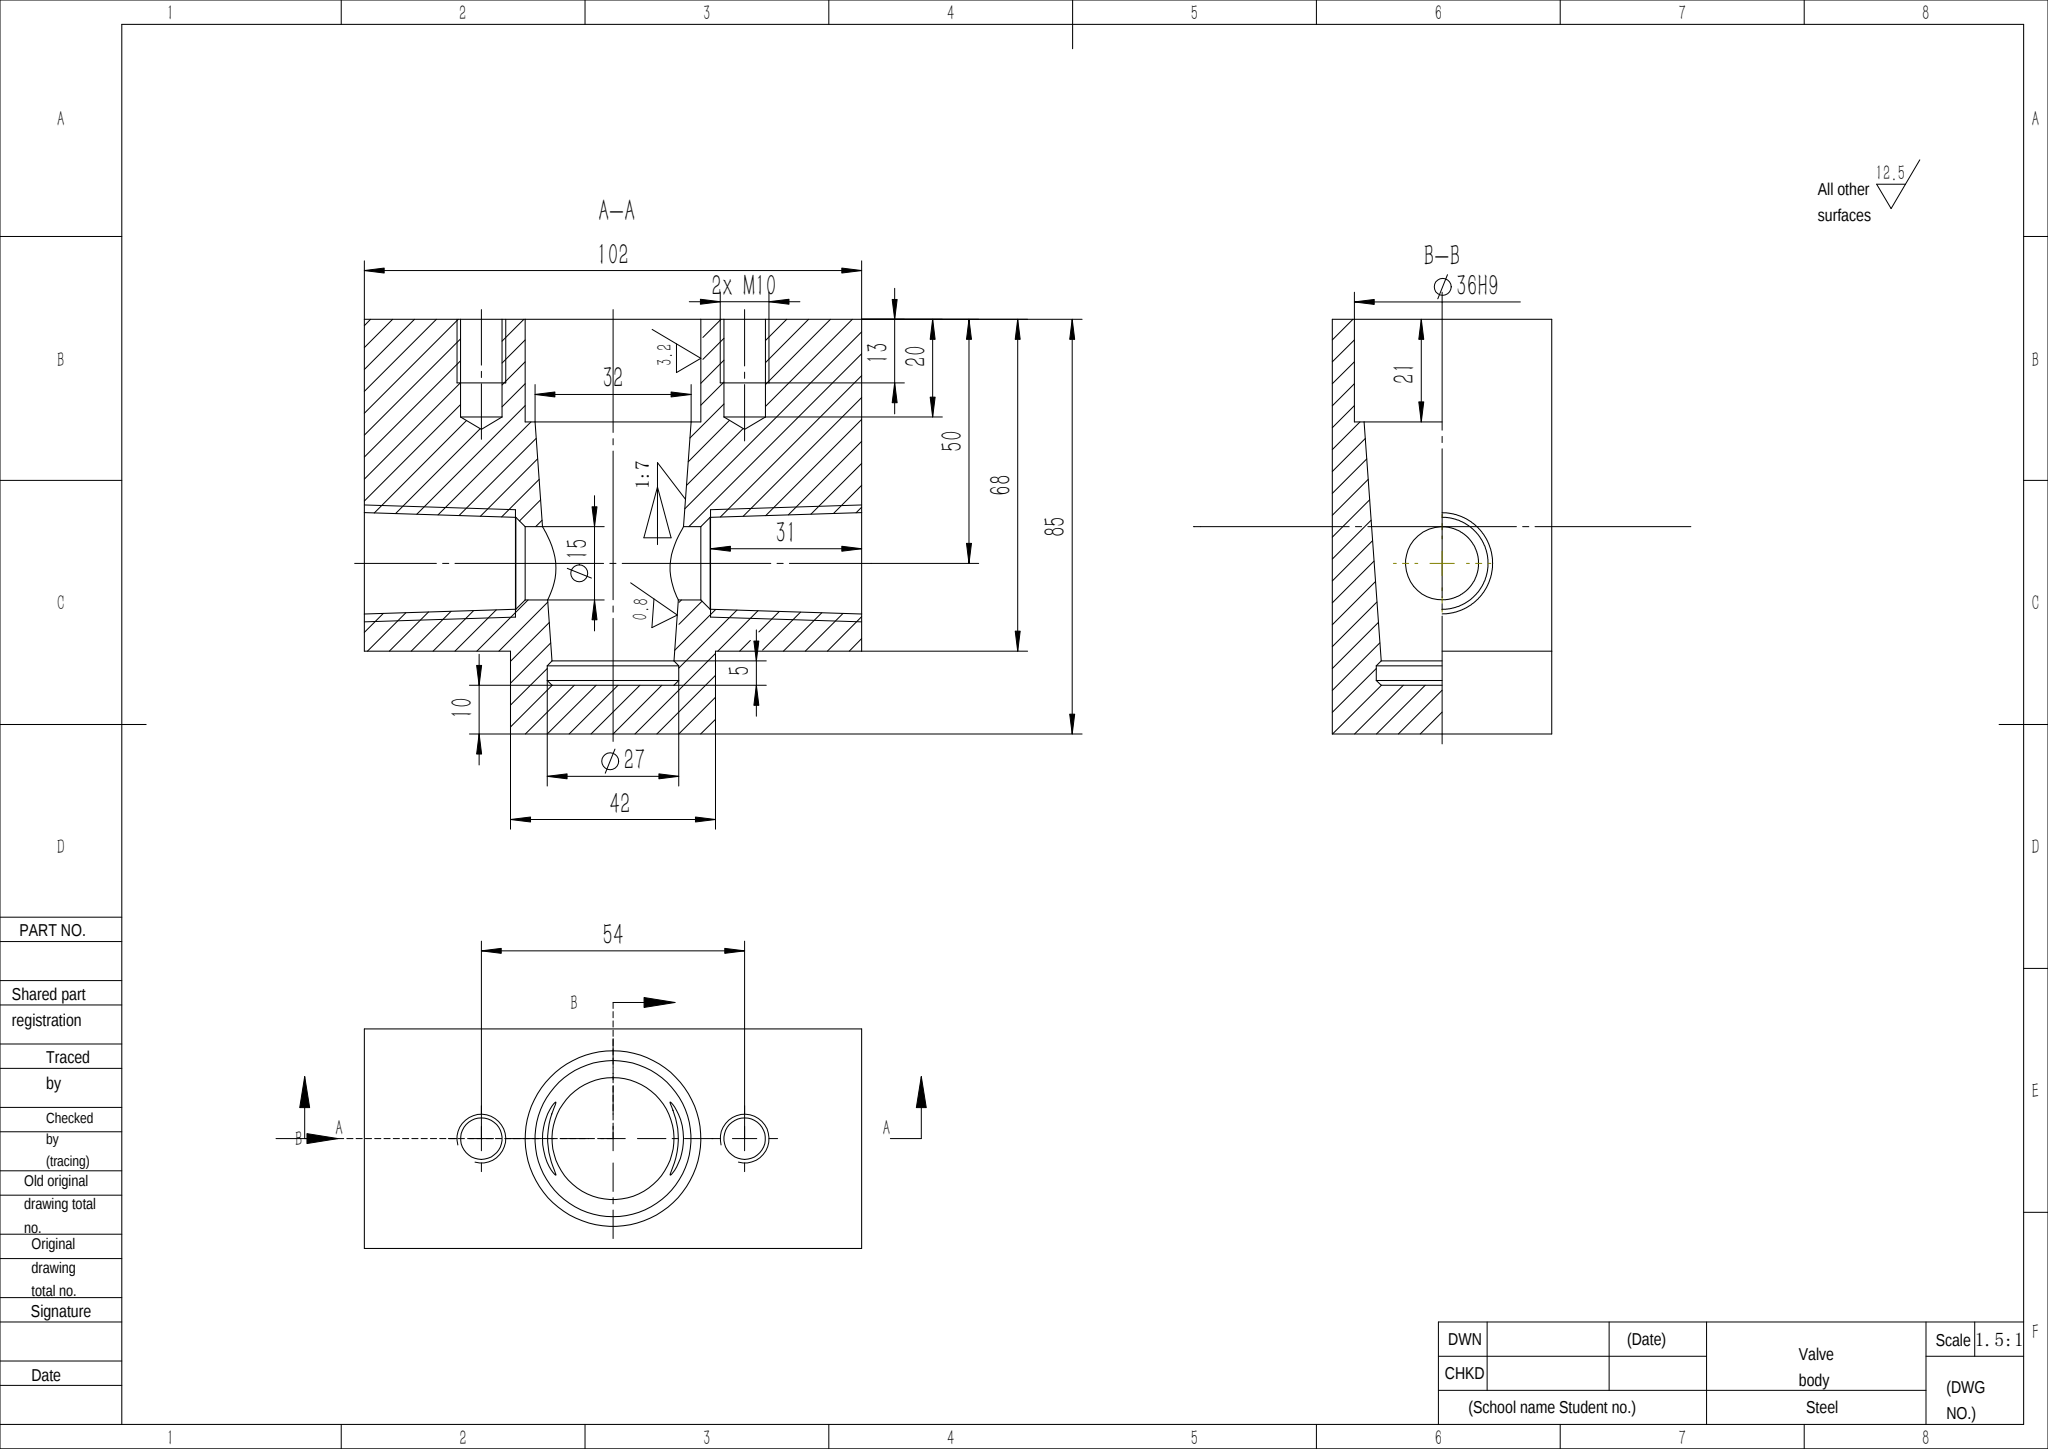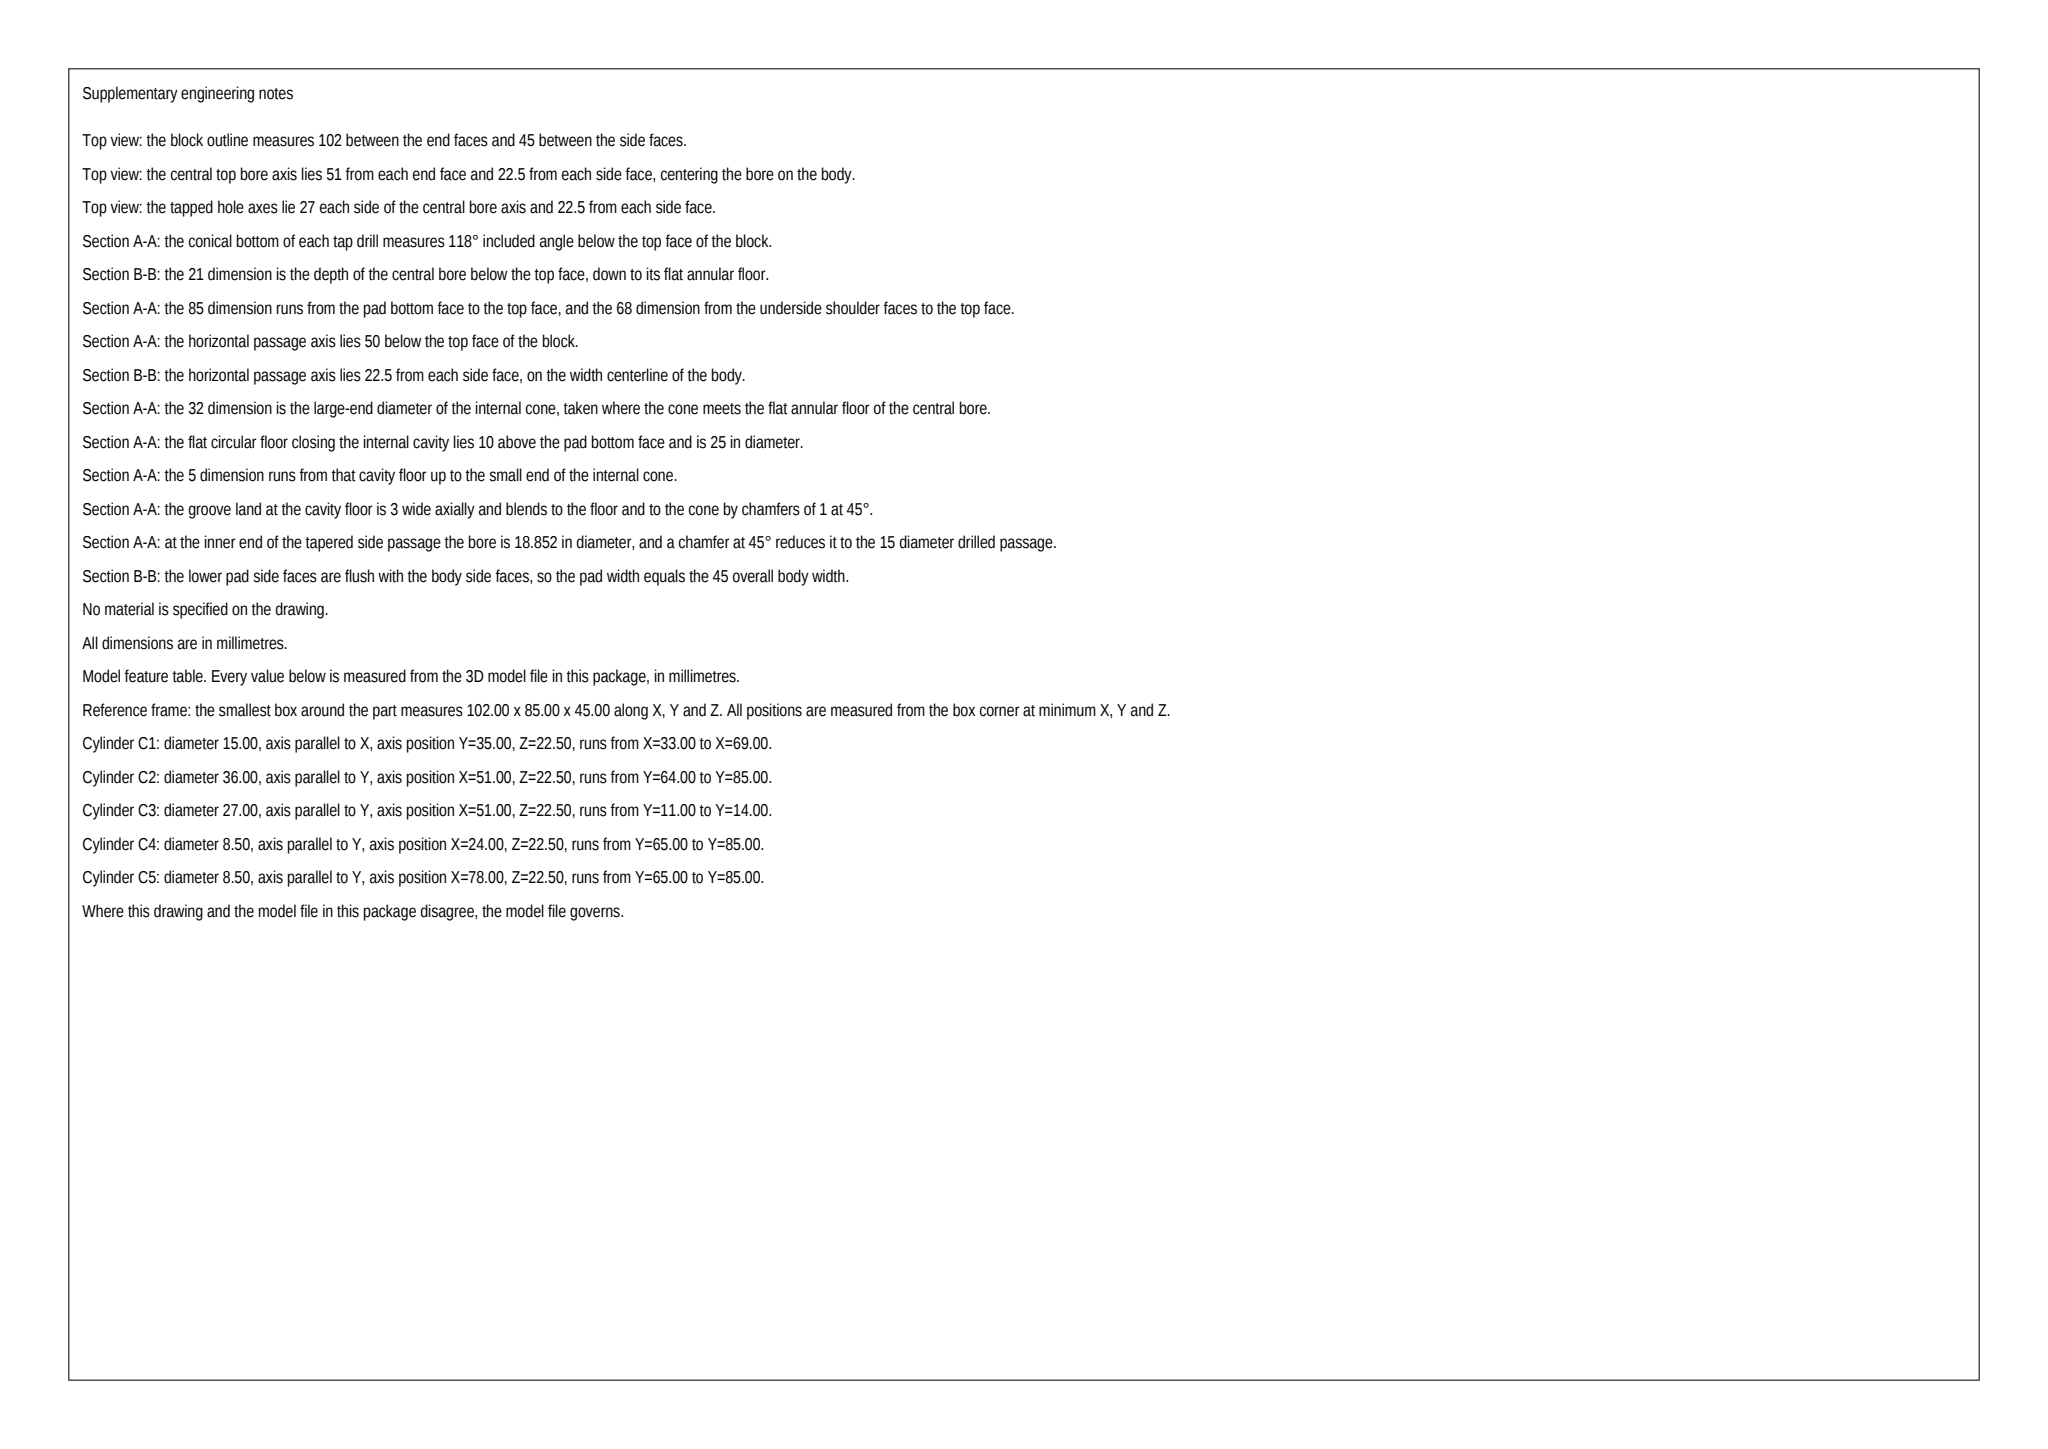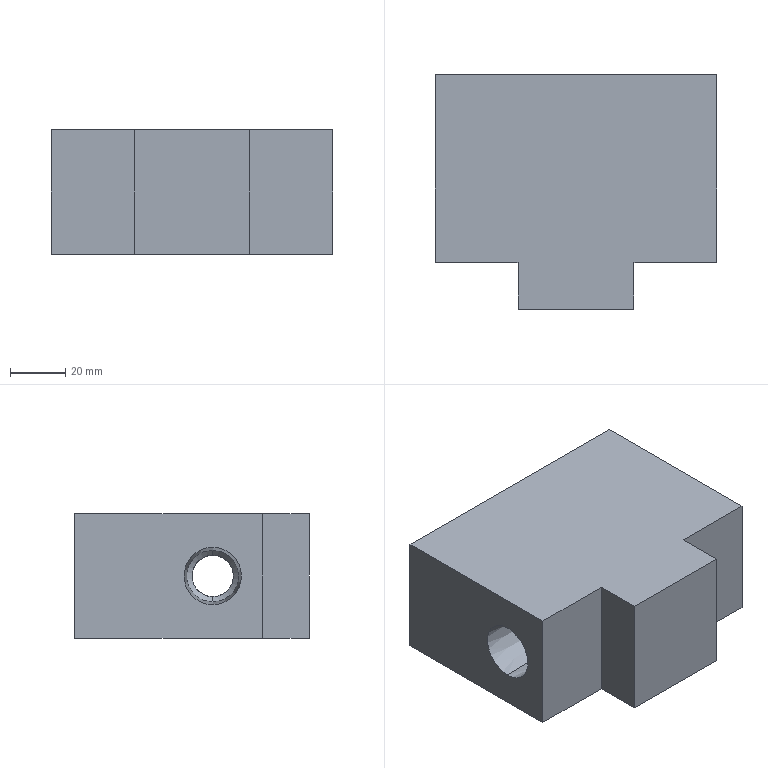Part | SolidWorks | mm | 1 solid | 42 faces | box 102 x 85 x 45 mm | volume 264623 mm3 | cone 18 | cylinder 12 | plane 12 | commonest cylinder face diameters 15 x4 8.5 x4 27 x2 36 x2
Drawing notes:
BORE MOUTH CSK 90 DEG INCL AT Ø15, Ø25 & Ø27 (A-A) | from the solid: cones[included_angle,ref_dia]: [90.0,15.0]x4, [90.0,25.0]x2, [90.0,27.0]x2
1:7 TAPER SEAT: REF Ø25 AT HORIZ BORE C/L, 35 FROM BASE | from the solid: cone [8.2 deg incl, ref_dia 25.0]x2 = 1:7; bore axis y=35 of 85 bbox
END BORES TAPER 1:16: Ø20.8 AT FACE TO Ø18.9 AT 30 DEEP, 2X | from the solid: cone [3.6 deg incl, ref_dia 20.792]x4; x-planes 0/30 and 72/102 => 30 lg, (20.8-18.9)/30=1:16
Ø15 STRAIGHT BORE LG: 6.26 LH & 6.31 RH BTWN TAPER & CAVITY | from the solid: cylinders [15,x,[null,35,22.5],6.26] and [15,x,[null,35,22.5],6.31]